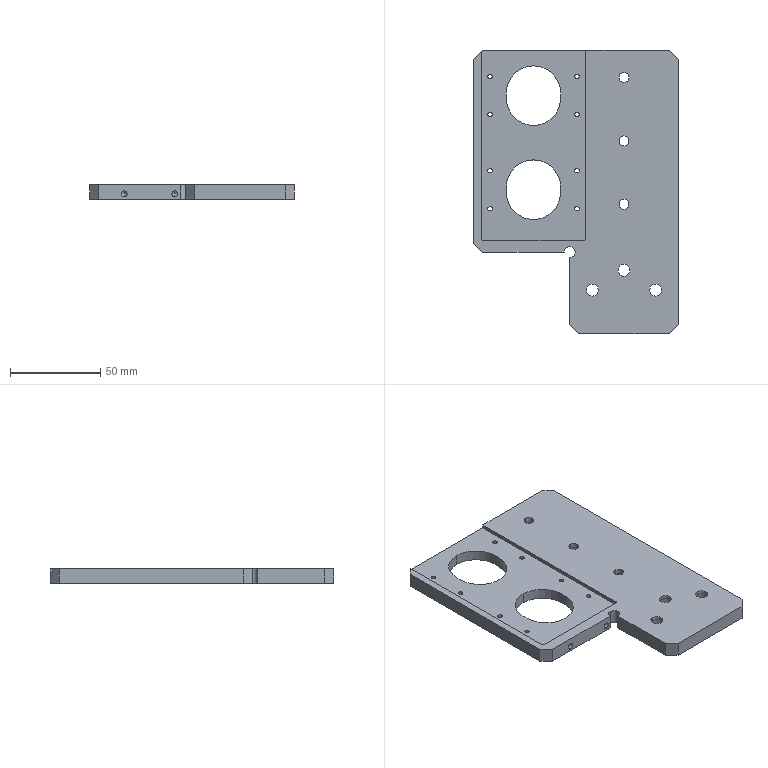Component | SolidWorks | 03-SmallMotorFixingPlate-1 | 1 solid | 93 faces | volume 96038 mm3 | cylinder 58 | plane 27 | cone 8 | commonest cylinder face diameters 2.5 x16 3.3 x8 30 x6 11 x6 6.6 x6 10 x6 5.5 x6 6 x2 | material Plain Carbon Steel